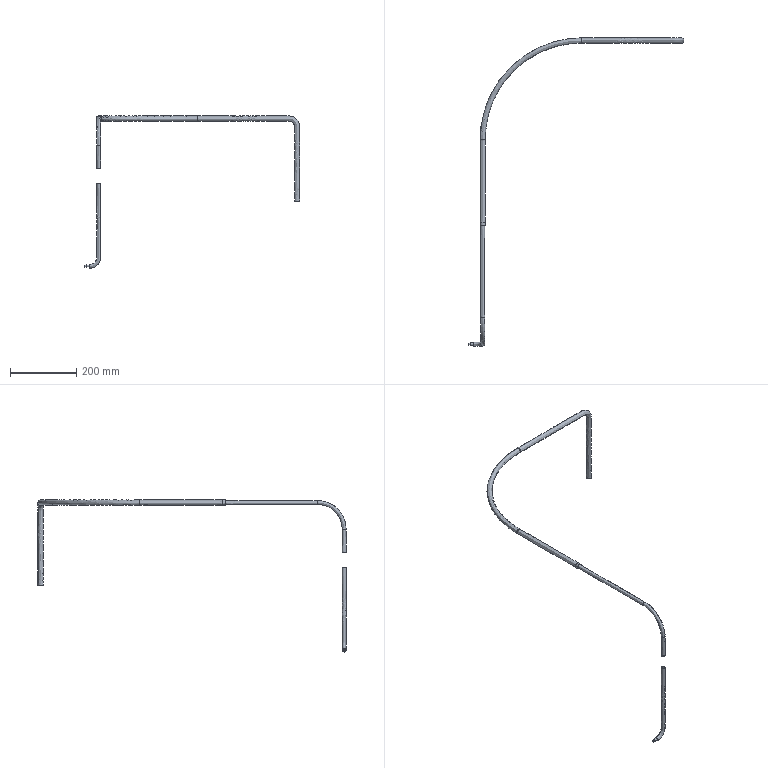Component | NX | WATER_PIPE | 4 solids | 27 faces | volume 152866 mm3 | spline 14 | plane 10 | cylinder 3 | commonest cylinder face diameters 12.04 x1 8.5 x1 5.96 x1